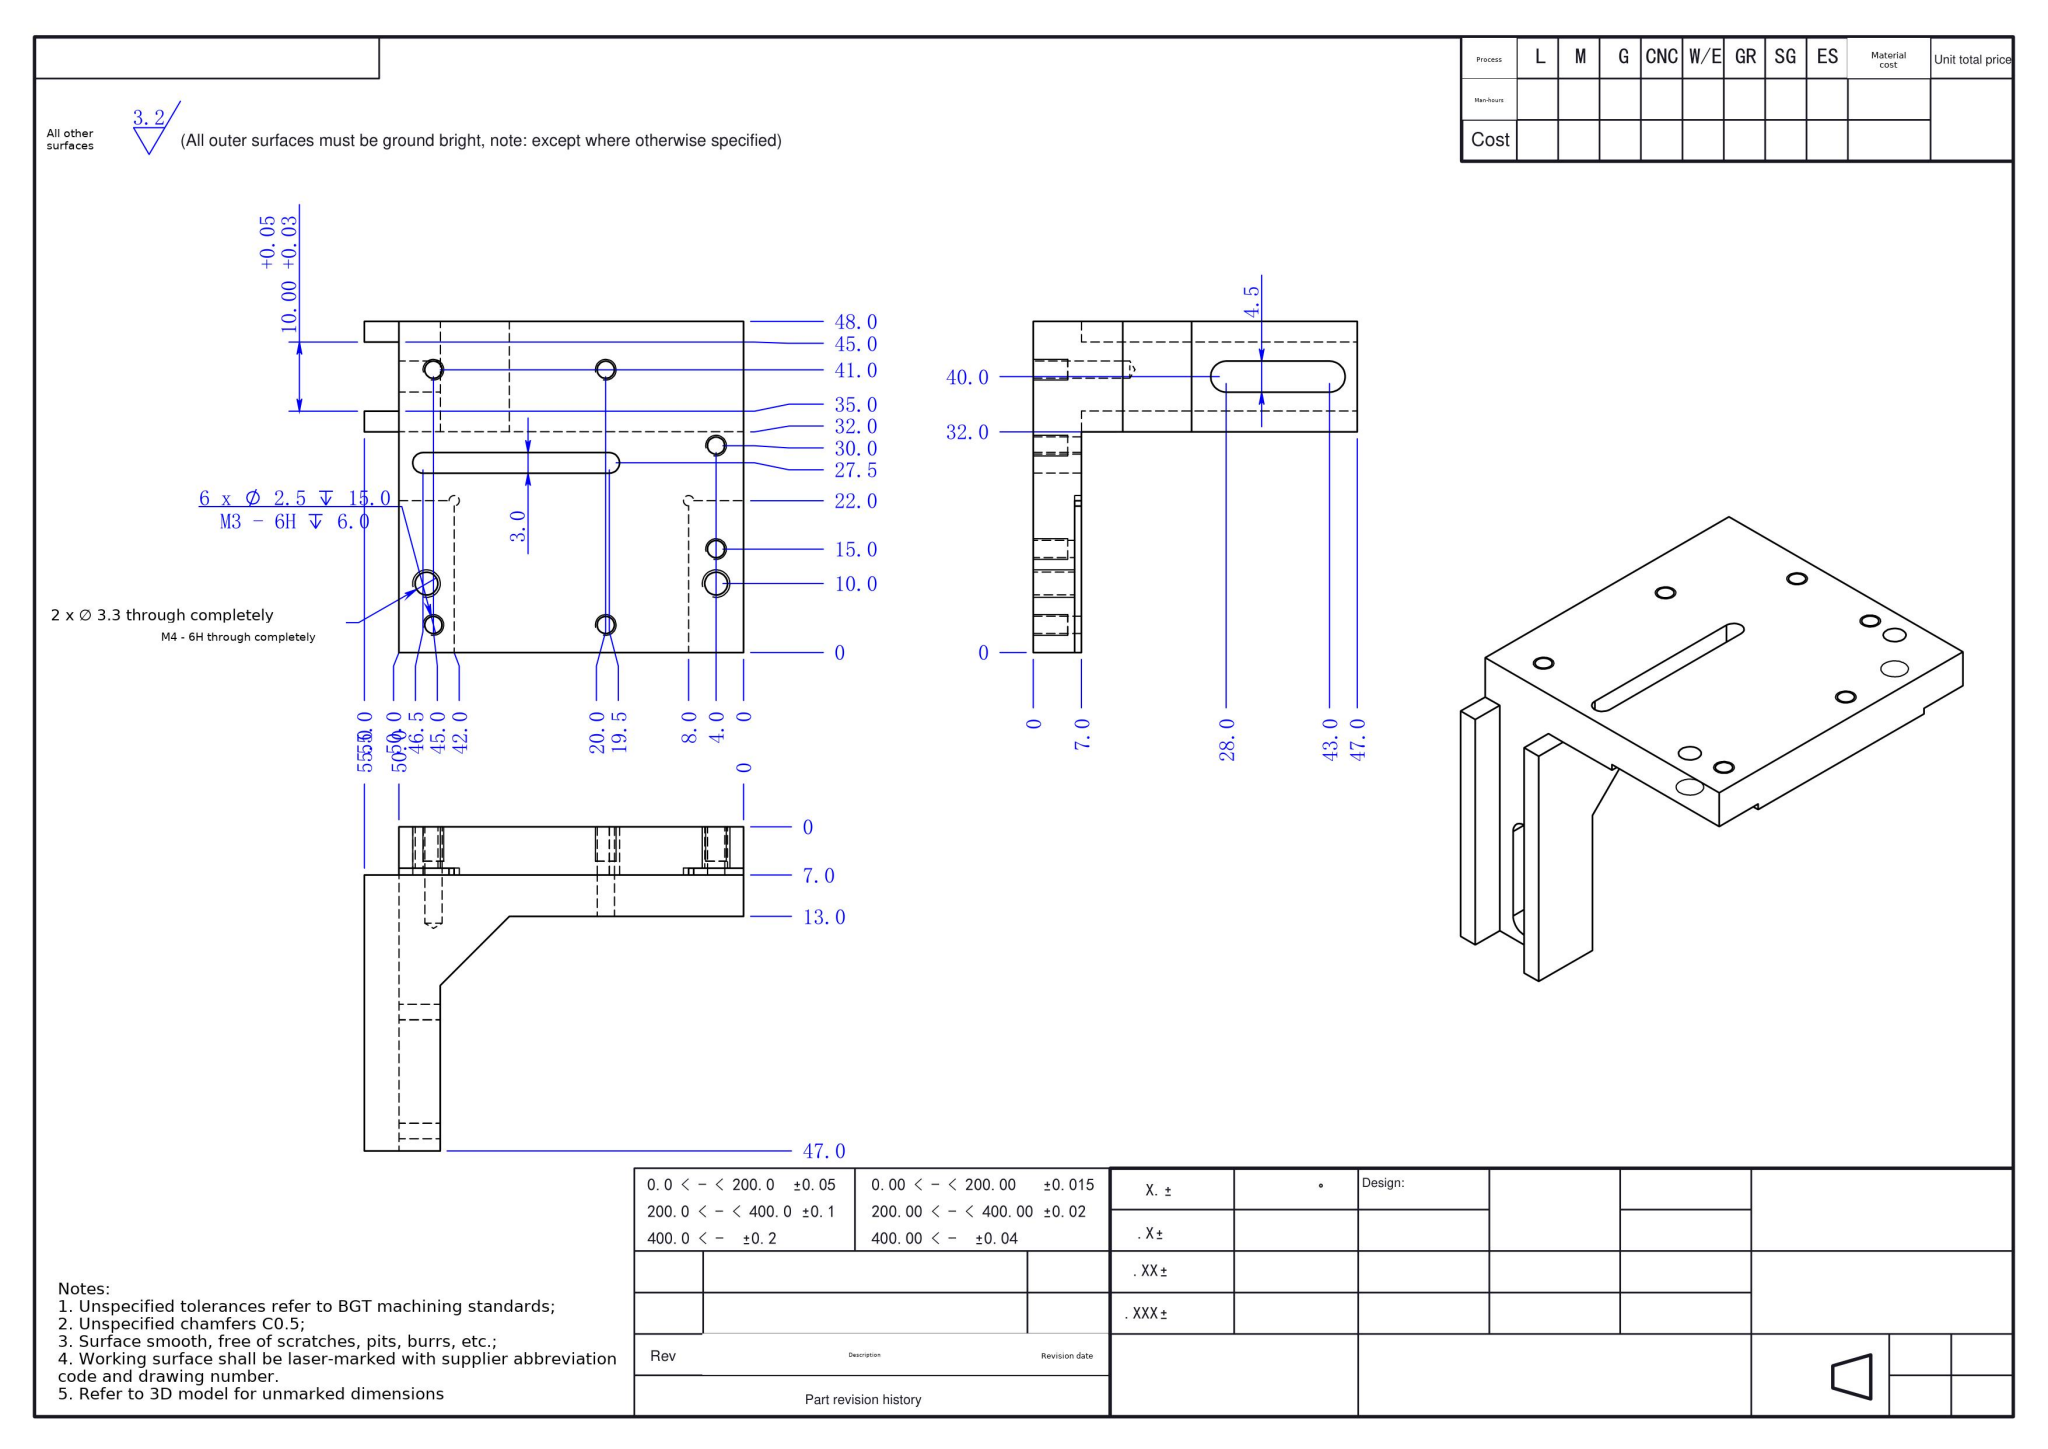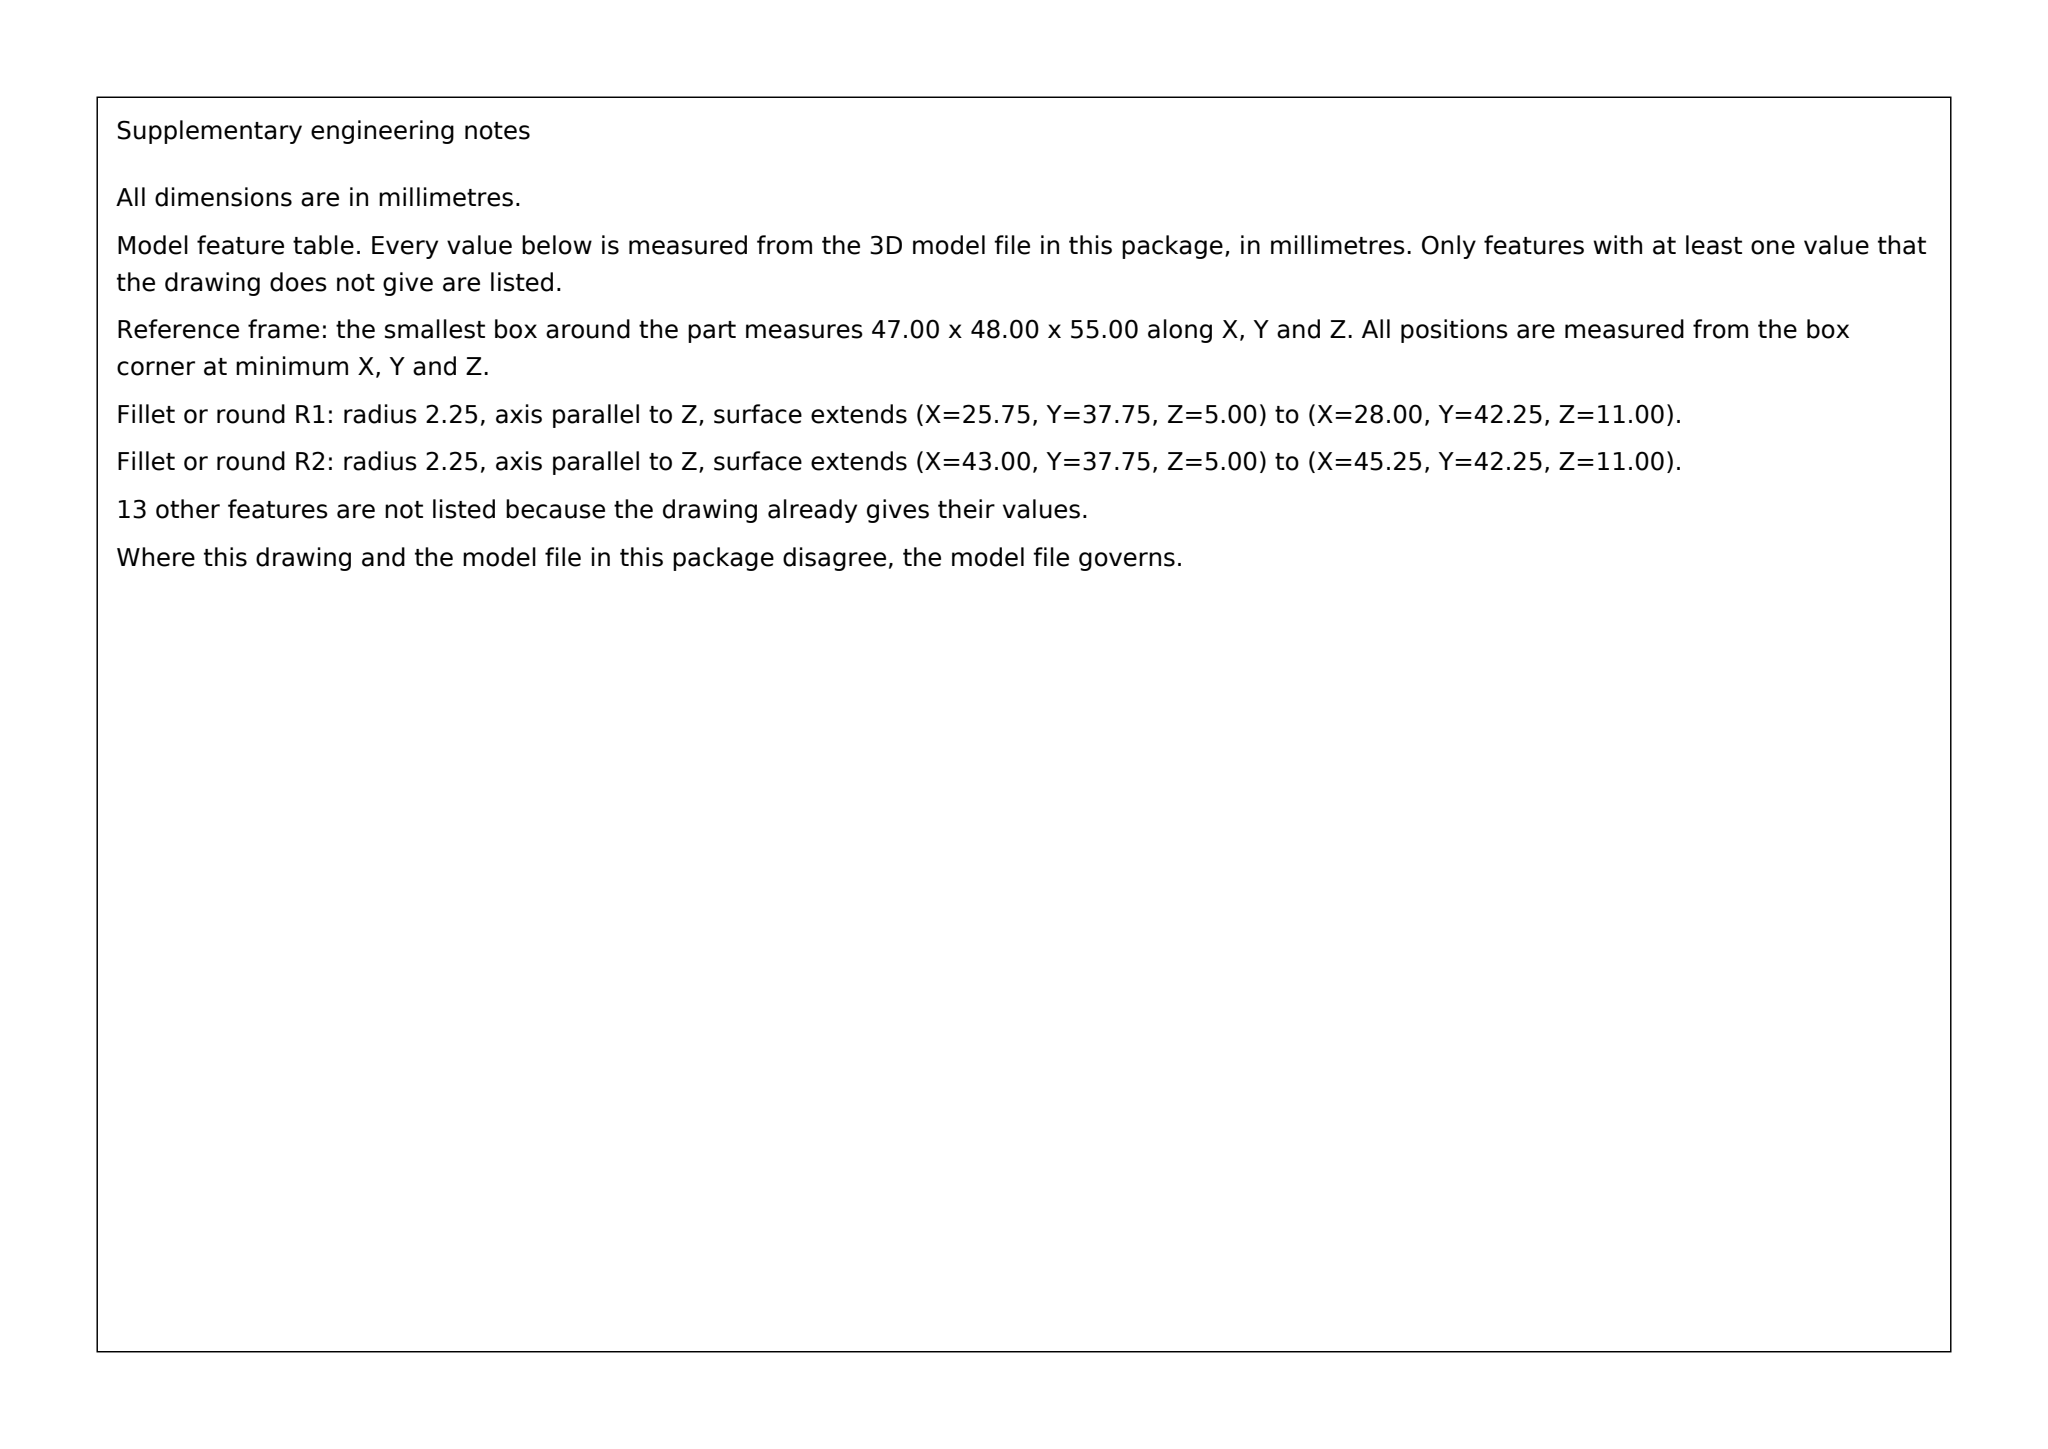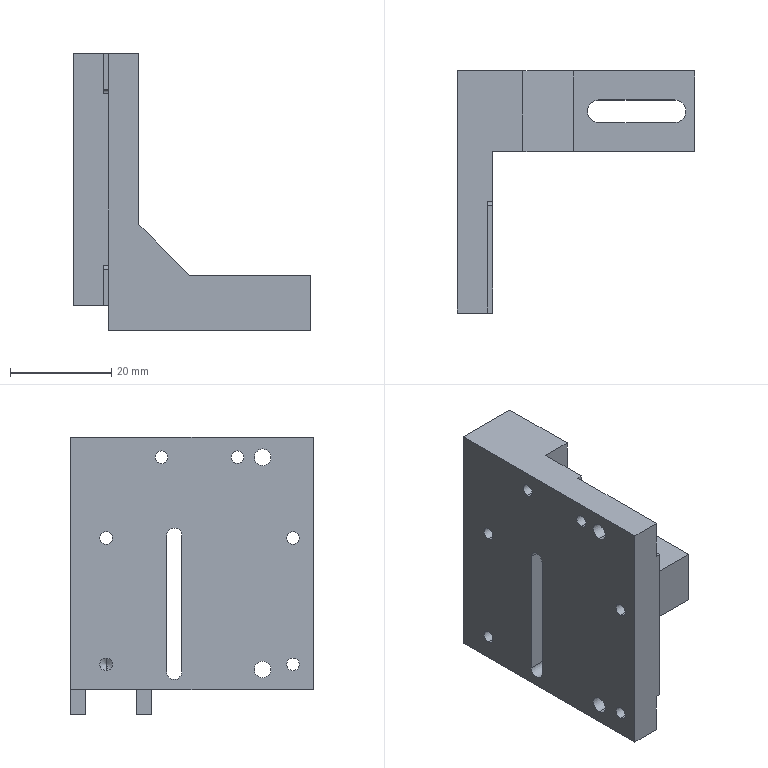Part | SolidWorks | mm | 1 solid | 54 faces | box 47 x 48 x 55 mm | volume 25028 mm3 | plane 27 | cylinder 25 | cone 2 | commonest cylinder face diameters 2.5 x12 3.3 x4 1.5 x3 3 x3 4.5 x3
build123d program:
from build123d import *

# Parameters (mm, degrees)
SKETCH1_W             = 40
SKETCH1_H             = 10
BOSS_EXTRUDE1_DEPTH   = 6
SKETCH2_W             = 6
SKETCH2_H             = 10
BOSS_EXTRUDE2_DEPTH   = 40
CHAMFER1_SIZE         = 10
SKETCH3_W             = 15.5
SKETCH3_H             = 10
BOSS_EXTRUDE4_DEPTH   = 8
CUT_EXTRUDE7_DEPTH    = 78.984
SKETCH10_W            = 8
SKETCH10_H            = 10
CUT_EXTRUDE8_DEPTH    = 5.5
SKETCH13_W            = 8
SKETCH13_H            = 46
BOSS_EXTRUDE5_DEPTH   = 45
BOSS_EXTRUDE6_DEPTH   = 4
SKETCH15_W            = 44
SKETCH15_H            = 31
CUT_EXTRUDE9_DEPTH    = 1
SKETCH18_W            = 40
SKETCH18_H            = 11
BOSS_EXTRUDE7_DEPTH   = 3
BOSS_EXTRUDE8_DEPTH   = 3
SKETCH20_R            = 1
CUT_EXTRUDE11_DEPTH   = 1
M3_TAPPED_HOLE1_D     = 2.5
M3_TAPPED_HOLE1_DEPTH = 15
M3_TAPPED_HOLE1_TIP   = 0.7511
CUT_EXTRUDE10_DEPTH   = 83.061
M4_TAPPED_HOLE1_D     = 3.3
BOSS_EXTRUDE10_DEPTH  = 3
SKETCH29_W            = 8
SKETCH29_H            = 22
CUT_EXTRUDE12_DEPTH   = 1
SKETCH30_R            = 0.75
CUT_EXTRUDE13_DEPTH   = 1
SKETCH31_W            = 1
SKETCH31_H            = 50
CUT_EXTRUDE14_DEPTH   = 96.841


with BuildPart() as part:
    # Sketch1 → Boss-Extrude1 (new body)
    with BuildSketch(Plane.XY):
        with Locations((46.193, -5)):
            Rectangle(SKETCH1_W, SKETCH1_H)
    extrude(amount=BOSS_EXTRUDE1_DEPTH)

    # Sketch2 → Boss-Extrude2 (add)
    with BuildSketch(Plane.XY.offset(6)):
        with Locations((29.193, -5)):
            Rectangle(SKETCH2_W, SKETCH2_H)
    extrude(amount=BOSS_EXTRUDE2_DEPTH)

    # Chamfer1
    chamfer1_edges = [part.edges().sort_by_distance(p)[0] for p in [
        (32.193, -5, 6),
    ]]
    chamfer(chamfer1_edges, length=CHAMFER1_SIZE)

    # Sketch3 → Boss-Extrude4 (add)
    with BuildSketch(Plane.ZY.offset(-26.193)):
        with Locations((7.75, -5)):
            Rectangle(SKETCH3_W, SKETCH3_H)
    extrude(amount=BOSS_EXTRUDE4_DEPTH)

    # Sketch9 → Cut-Extrude7 (cut, through all)
    with BuildSketch(Plane.XY.offset(6)):
        with BuildLine():
            Line((62.193, -7.25), (47.193, -7.25))
            ThreePointArc((47.193, -7.25), (44.943, -5), (47.193, -2.75))
            Line((47.193, -2.75), (62.193, -2.75))
            ThreePointArc((62.193, -2.75), (64.443, -5), (62.193, -7.25))
        make_face()
    extrude(amount=-CUT_EXTRUDE7_DEPTH, mode=Mode.SUBTRACT)

    # Sketch10 → Cut-Extrude8 (cut)
    with BuildSketch(Plane.XY.offset(15.5)):
        with Locations((22.193, -5)):
            Rectangle(SKETCH10_W, SKETCH10_H)
    extrude(amount=-CUT_EXTRUDE8_DEPTH, mode=Mode.SUBTRACT)

    # Sketch13 → Boss-Extrude5 (add)
    with BuildSketch(Plane(origin=(0, 0, 0), x_dir=(1, 0, 0), z_dir=(0, 1, 0))):
        with Locations((22.193, -23)):
            Rectangle(SKETCH13_W, SKETCH13_H)
    extrude(amount=-BOSS_EXTRUDE5_DEPTH)

    # Sketch14 → Boss-Extrude6 (add)
    with BuildSketch(Plane.XY.offset(46)):
        Polygon((32.193, 0), (18.193, 0), (18.193, -45), (26.193, -45), (26.193, -10), (32.193, -10), align=None)
    extrude(amount=BOSS_EXTRUDE6_DEPTH)

    # Sketch15 → Cut-Extrude9 (cut)
    with BuildSketch(Plane.ZY.offset(-18.193)):
        with Locations((22, -23.5)):
            Rectangle(SKETCH15_W, SKETCH15_H)
    extrude(amount=-CUT_EXTRUDE9_DEPTH, mode=Mode.SUBTRACT)

    # Sketch18 → Boss-Extrude7 (add)
    with BuildSketch(Plane.XZ.offset(10)):
        with Locations((46.193, 0.5)):
            Rectangle(SKETCH18_W, SKETCH18_H)
    extrude(amount=BOSS_EXTRUDE7_DEPTH)

    # Sketch19 → Boss-Extrude8 (add)
    with BuildSketch(Plane.XZ.offset(10)):
        Polygon((26.193, 6), (42.193, 6), (32.193, 16), (32.193, 50), (26.193, 50), align=None)
    extrude(amount=BOSS_EXTRUDE8_DEPTH)

    # Sketch20 → Cut-Extrude11 (cut)
    with BuildSketch(Plane.ZY.offset(-18.193)):
        with Locations((44, -8)):
            Circle(SKETCH20_R)
        with Locations((44, -39)):
            Circle(SKETCH20_R)
    extrude(amount=-CUT_EXTRUDE11_DEPTH, mode=Mode.SUBTRACT)

    # M3 Tapped Hole1
    with Locations(Plane.ZY.offset(-18.193)):
        with Locations((5, -4), (30, -4), (46, -15), (46, -30), (30, -41), (5, -41)):
            Hole(M3_TAPPED_HOLE1_D / 2, depth=M3_TAPPED_HOLE1_DEPTH)
            with Locations((0, 0, -(M3_TAPPED_HOLE1_DEPTH + M3_TAPPED_HOLE1_TIP / 2))):  # 118° drill point
                Cone(0, M3_TAPPED_HOLE1_D / 2, M3_TAPPED_HOLE1_TIP, mode=Mode.SUBTRACT)

    # Sketch16 → Cut-Extrude10 (cut, through all)
    with BuildSketch(Plane.ZY.offset(-19.193)):
        with BuildLine():
            Line((30.5, -19), (3.5, -19))
            ThreePointArc((3.5, -19), (2, -17.5), (3.5, -16))
            Line((3.5, -16), (30.5, -16))
            ThreePointArc((30.5, -16), (32, -17.5), (30.5, -19))
        make_face()
    extrude(amount=-CUT_EXTRUDE10_DEPTH, mode=Mode.SUBTRACT)

    # M4 Tapped Hole1 (through all)
    with Locations(Plane(origin=(26.193, 0, 0), x_dir=(0, 0, -1), z_dir=(1, 0, 0))):
        with Locations((-4, -35), (-46, -35)):
            Hole(M4_TAPPED_HOLE1_D / 2)

    # Sketch28 → Boss-Extrude10 (add)
    with BuildSketch(Plane(origin=(0, 0, 0), x_dir=(1, 0, 0), z_dir=(0, 1, 0))):
        Polygon((26.193, 0), (18.193, 0), (18.193, -50), (32.193, -50), (32.193, -16), (42.193, -6), (66.193, -6), (66.193, 0), (66.193, 5), (26.193, 5), align=None)
    extrude(amount=BOSS_EXTRUDE10_DEPTH)

    # Sketch29 → Cut-Extrude12 (cut)
    with BuildSketch(Plane(origin=(26.193, 0, 0), x_dir=(0, 0, -1), z_dir=(1, 0, 0))):
        with Locations((-46, -34)):
            Rectangle(SKETCH29_W, SKETCH29_H)
        with Locations((-4, -34)):
            Rectangle(SKETCH29_W, SKETCH29_H)
    extrude(amount=-CUT_EXTRUDE12_DEPTH, mode=Mode.SUBTRACT)

    # Sketch30 → Cut-Extrude13 (cut)
    with BuildSketch(Plane(origin=(26.193, 0, 0), x_dir=(0, 0, -1), z_dir=(1, 0, 0))):
        with Locations((-42, -23)):
            Circle(SKETCH30_R)
        with Locations((-8, -23)):
            Circle(SKETCH30_R)
    extrude(amount=-CUT_EXTRUDE13_DEPTH, mode=Mode.SUBTRACT)

    # Sketch31 → Cut-Extrude14 (cut, through all)
    with BuildSketch(Plane.XZ.offset(45)):
        with Locations((18.693, 25)):
            Rectangle(SKETCH31_W, SKETCH31_H)
    extrude(amount=-CUT_EXTRUDE14_DEPTH, mode=Mode.SUBTRACT)


solid = part.part